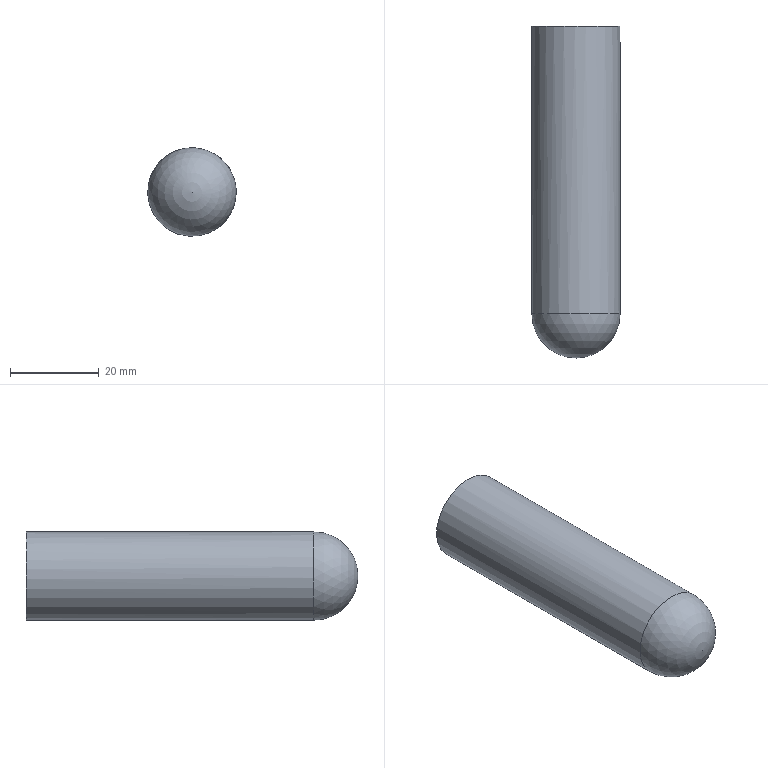Component | NX | PLUNGER_2 | 1 solid | 5 faces | box 20 x 75 x 20 mm | volume 9446 mm3 | cylinder 2 | plane 2 | sphere 1 | commonest cylinder face diameters 20 x1 16 x1
STEP:
#1=CARTESIAN_POINT('',(0.,0.,0.));
#2=DIRECTION('',(0.,0.,1.));
#3=DIRECTION('',(1.,0.,0.));
#4=AXIS2_PLACEMENT_3D('',#1,#2,#3);
#5=CARTESIAN_POINT('',(-34.641,119.,-20.));
#6=VERTEX_POINT('',#5);
#7=CARTESIAN_POINT('',(-17.321,119.,-10.));
#8=VERTEX_POINT('',#7);
#9=CARTESIAN_POINT('',(-25.981,119.,-15.));
#10=DIRECTION('',(0.,1.,0.));
#11=DIRECTION('',(-0.866,0.,-0.5));
#12=AXIS2_PLACEMENT_3D('',#9,#10,#11);
#13=CIRCLE('',#12,10.);
#14=CARTESIAN_POINT('',(-25.981,109.,-15.));
#15=DIRECTION('',(0.,1.,0.));
#16=DIRECTION('',(-0.866,0.,-0.5));
#17=AXIS2_PLACEMENT_3D('',#14,#15,#16);
#18=CYLINDRICAL_SURFACE('',#17,10.);
#19=CARTESIAN_POINT('',(0.,10.));
#20=DIRECTION('',(1.,0.));
#21=VECTOR('',#20,1.);
#22=LINE('',#19,#21);
#23=(GEOMETRIC_REPRESENTATION_CONTEXT(2)PARAMETRIC_REPRESENTATION_CONTEXT()REPRESENTATION_CONTEXT('',''));
#24=DEFINITIONAL_REPRESENTATION('',(#22),#23);
#25=PCURVE('',#18,#24);
#26=CARTESIAN_POINT('',(-25.981,119.,-15.));
#27=DIRECTION('',(0.,-1.,0.));
#28=DIRECTION('',(0.866,0.,0.5));
#29=AXIS2_PLACEMENT_3D('',#26,#27,#28);
#30=SPHERICAL_SURFACE('',#29,10.);
#31=CARTESIAN_POINT('',(3.142,0.));
#32=CARTESIAN_POINT('',(3.046,0.));
#33=CARTESIAN_POINT('',(2.856,0.));
#34=CARTESIAN_POINT('',(2.57,0.));
#35=CARTESIAN_POINT('',(2.285,0.));
#36=CARTESIAN_POINT('',(1.999,0.));
#37=CARTESIAN_POINT('',(1.714,0.));
#38=CARTESIAN_POINT('',(1.428,0.));
#39=CARTESIAN_POINT('',(1.142,0.));
#40=CARTESIAN_POINT('',(0.8568,0.));
#41=CARTESIAN_POINT('',(0.5712,0.));
#42=CARTESIAN_POINT('',(0.2856,0.));
#43=CARTESIAN_POINT('',(0.,0.));
#44=CARTESIAN_POINT('',(-0.2856,0.));
#45=CARTESIAN_POINT('',(-0.5712,0.));
#46=CARTESIAN_POINT('',(-0.8568,0.));
#47=CARTESIAN_POINT('',(-1.142,0.));
#48=CARTESIAN_POINT('',(-1.428,0.));
#49=CARTESIAN_POINT('',(-1.714,0.));
#50=CARTESIAN_POINT('',(-1.999,0.));
#51=CARTESIAN_POINT('',(-2.285,0.));
#52=CARTESIAN_POINT('',(-2.57,0.));
#53=CARTESIAN_POINT('',(-2.856,0.));
#54=CARTESIAN_POINT('',(-3.046,0.));
#55=CARTESIAN_POINT('',(-3.142,0.));
#56=B_SPLINE_CURVE_WITH_KNOTS('',3,(#31,#32,#33,#34,#35,#36,#37,#38,#39,#40,#41,#42,#43,#44,#45,#46,#47,#48,#49,#50,#51,#52,#53,#54,#55),.UNSPECIFIED.,.F.,.F.,(4,1,1,1,1,1,1,1,1,1,1,1,1,1,1,1,1,1,1,1,1,1,4),(0.,0.2856,0.5712,0.8568,1.142,1.428,1.714,1.999,2.285,2.57,2.856,3.142,3.427,3.713,3.998,4.284,4.57,4.855,5.141,5.426,5.712,5.998,6.283),.QUASI_UNIFORM_KNOTS.);
#57=(GEOMETRIC_REPRESENTATION_CONTEXT(2)PARAMETRIC_REPRESENTATION_CONTEXT()REPRESENTATION_CONTEXT('',''));
#58=DEFINITIONAL_REPRESENTATION('',(#56),#57);
#59=PCURVE('',#30,#58);
#60=SURFACE_CURVE('',#13,(#25,#59),.PCURVE_S1.);
#61=EDGE_CURVE('',#6,#8,#60,.T.);
#62=ORIENTED_EDGE('',*,*,#61,.T.);
#63=CARTESIAN_POINT('',(-25.981,119.,-15.));
#64=DIRECTION('',(0.,1.,0.));
#65=DIRECTION('',(-0.866,0.,-0.5));
#66=AXIS2_PLACEMENT_3D('',#63,#64,#65);
#67=CIRCLE('',#66,10.);
#68=CARTESIAN_POINT('',(0.,10.));
#69=DIRECTION('',(1.,0.));
#70=VECTOR('',#69,1.);
#71=LINE('',#68,#70);
#72=(GEOMETRIC_REPRESENTATION_CONTEXT(2)PARAMETRIC_REPRESENTATION_CONTEXT()REPRESENTATION_CONTEXT('',''));
#73=DEFINITIONAL_REPRESENTATION('',(#71),#72);
#74=PCURVE('',#18,#73);
#75=CARTESIAN_POINT('',(9.425,0.));
#76=CARTESIAN_POINT('',(9.33,0.));
#77=CARTESIAN_POINT('',(9.139,0.));
#78=CARTESIAN_POINT('',(8.854,0.));
#79=CARTESIAN_POINT('',(8.568,0.));
#80=CARTESIAN_POINT('',(8.282,0.));
#81=CARTESIAN_POINT('',(7.997,0.));
#82=CARTESIAN_POINT('',(7.711,0.));
#83=CARTESIAN_POINT('',(7.426,0.));
#84=CARTESIAN_POINT('',(7.14,0.));
#85=CARTESIAN_POINT('',(6.854,0.));
#86=CARTESIAN_POINT('',(6.569,0.));
#87=CARTESIAN_POINT('',(6.283,0.));
#88=CARTESIAN_POINT('',(5.998,0.));
#89=CARTESIAN_POINT('',(5.712,0.));
#90=CARTESIAN_POINT('',(5.426,0.));
#91=CARTESIAN_POINT('',(5.141,0.));
#92=CARTESIAN_POINT('',(4.855,0.));
#93=CARTESIAN_POINT('',(4.57,0.));
#94=CARTESIAN_POINT('',(4.284,0.));
#95=CARTESIAN_POINT('',(3.998,0.));
#96=CARTESIAN_POINT('',(3.713,0.));
#97=CARTESIAN_POINT('',(3.427,0.));
#98=CARTESIAN_POINT('',(3.237,0.));
#99=CARTESIAN_POINT('',(3.142,0.));
#100=B_SPLINE_CURVE_WITH_KNOTS('',3,(#75,#76,#77,#78,#79,#80,#81,#82,#83,#84,#85,#86,#87,#88,#89,#90,#91,#92,#93,#94,#95,#96,#97,#98,#99),.UNSPECIFIED.,.F.,.F.,(4,1,1,1,1,1,1,1,1,1,1,1,1,1,1,1,1,1,1,1,1,1,4),(0.,0.2856,0.5712,0.8568,1.142,1.428,1.714,1.999,2.285,2.57,2.856,3.142,3.427,3.713,3.998,4.284,4.57,4.855,5.141,5.426,5.712,5.998,6.283),.QUASI_UNIFORM_KNOTS.);
#101=(GEOMETRIC_REPRESENTATION_CONTEXT(2)PARAMETRIC_REPRESENTATION_CONTEXT()REPRESENTATION_CONTEXT('',''));
#102=DEFINITIONAL_REPRESENTATION('',(#100),#101);
#103=PCURVE('',#30,#102);
#104=SURFACE_CURVE('',#67,(#74,#103),.PCURVE_S1.);
#105=EDGE_CURVE('',#8,#6,#104,.T.);
#106=ORIENTED_EDGE('',*,*,#105,.T.);
#107=CARTESIAN_POINT('',(-34.641,184.,-20.));
#108=VERTEX_POINT('',#107);
#109=CARTESIAN_POINT('',(-34.641,119.,-20.));
#110=CARTESIAN_POINT('',(-34.641,184.,-20.));
#111=B_SPLINE_CURVE_WITH_KNOTS('',1,(#109,#110),.UNSPECIFIED.,.F.,.F.,(2,2),(10.,75.),.PIECEWISE_BEZIER_KNOTS.);
#112=CARTESIAN_POINT('',(6.283,0.));
#113=DIRECTION('',(0.,1.));
#114=VECTOR('',#113,1.);
#115=LINE('',#112,#114);
#116=(GEOMETRIC_REPRESENTATION_CONTEXT(2)PARAMETRIC_REPRESENTATION_CONTEXT()REPRESENTATION_CONTEXT('',''));
#117=DEFINITIONAL_REPRESENTATION('',(#115),#116);
#118=PCURVE('',#18,#117);
#119=CARTESIAN_POINT('',(0.,0.));
#120=DIRECTION('',(0.,1.));
#121=VECTOR('',#120,1.);
#122=LINE('',#119,#121);
#123=(GEOMETRIC_REPRESENTATION_CONTEXT(2)PARAMETRIC_REPRESENTATION_CONTEXT()REPRESENTATION_CONTEXT('',''));
#124=DEFINITIONAL_REPRESENTATION('',(#122),#123);
#125=PCURVE('',#18,#124);
#126=SEAM_CURVE('',#111,(#118,#125),.PCURVE_S1.);
#127=EDGE_CURVE('',#6,#108,#126,.T.);
#128=ORIENTED_EDGE('',*,*,#127,.T.);
#129=CARTESIAN_POINT('',(-30.981,184.,-6.34));
#130=VERTEX_POINT('',#129);
#131=CARTESIAN_POINT('',(-25.981,184.,-15.));
#132=DIRECTION('',(0.,-1.,0.));
#133=DIRECTION('',(-0.5,0.,0.866));
#134=AXIS2_PLACEMENT_3D('',#131,#132,#133);
#135=CIRCLE('',#134,10.);
#136=CARTESIAN_POINT('',(7.854,75.));
#137=DIRECTION('',(-1.,0.));
#138=VECTOR('',#137,1.);
#139=LINE('',#136,#138);
#140=(GEOMETRIC_REPRESENTATION_CONTEXT(2)PARAMETRIC_REPRESENTATION_CONTEXT()REPRESENTATION_CONTEXT('',''));
#141=DEFINITIONAL_REPRESENTATION('',(#139),#140);
#142=PCURVE('',#18,#141);
#143=CARTESIAN_POINT('',(-25.981,184.,-15.));
#144=DIRECTION('',(0.,-1.,0.));
#145=DIRECTION('',(0.866,0.,0.5));
#146=AXIS2_PLACEMENT_3D('',#143,#144,#145);
#147=PLANE('',#146);
#148=CARTESIAN_POINT('',(0.,0.));
#149=DIRECTION('',(0.,1.));
#150=AXIS2_PLACEMENT_2D('',#148,#149);
#151=CIRCLE('',#150,10.);
#152=(GEOMETRIC_REPRESENTATION_CONTEXT(2)PARAMETRIC_REPRESENTATION_CONTEXT()REPRESENTATION_CONTEXT('',''));
#153=DEFINITIONAL_REPRESENTATION('',(#151),#152);
#154=PCURVE('',#147,#153);
#155=SURFACE_CURVE('',#135,(#142,#154),.PCURVE_S1.);
#156=EDGE_CURVE('',#108,#130,#155,.T.);
#157=ORIENTED_EDGE('',*,*,#156,.T.);
#158=CARTESIAN_POINT('',(-25.981,184.,-15.));
#159=DIRECTION('',(0.,-1.,0.));
#160=DIRECTION('',(-0.5,0.,0.866));
#161=AXIS2_PLACEMENT_3D('',#158,#159,#160);
#162=CIRCLE('',#161,10.);
#163=CARTESIAN_POINT('',(1.571,75.));
#164=DIRECTION('',(-1.,0.));
#165=VECTOR('',#164,1.);
#166=LINE('',#163,#165);
#167=(GEOMETRIC_REPRESENTATION_CONTEXT(2)PARAMETRIC_REPRESENTATION_CONTEXT()REPRESENTATION_CONTEXT('',''));
#168=DEFINITIONAL_REPRESENTATION('',(#166),#167);
#169=PCURVE('',#18,#168);
#170=CARTESIAN_POINT('',(0.,0.));
#171=DIRECTION('',(0.,1.));
#172=AXIS2_PLACEMENT_2D('',#170,#171);
#173=CIRCLE('',#172,10.);
#174=(GEOMETRIC_REPRESENTATION_CONTEXT(2)PARAMETRIC_REPRESENTATION_CONTEXT()REPRESENTATION_CONTEXT('',''));
#175=DEFINITIONAL_REPRESENTATION('',(#173),#174);
#176=PCURVE('',#147,#175);
#177=SURFACE_CURVE('',#162,(#169,#176),.PCURVE_S1.);
#178=EDGE_CURVE('',#130,#108,#177,.T.);
#179=ORIENTED_EDGE('',*,*,#178,.T.);
#180=ORIENTED_EDGE('',*,*,#127,.F.);
#181=EDGE_LOOP('',(#62,#106,#128,#157,#179,#180));
#182=FACE_BOUND('',#181,.T.);
#183=ADVANCED_FACE('',(#182),#18,.T.);
#184=CARTESIAN_POINT('',(-19.053,184.,-11.));
#185=VERTEX_POINT('',#184);
#186=CARTESIAN_POINT('',(-25.981,184.,-15.));
#187=DIRECTION('',(0.,-1.,0.));
#188=DIRECTION('',(0.866,0.,0.5));
#189=AXIS2_PLACEMENT_3D('',#186,#187,#188);
#190=CIRCLE('',#189,8.);
#191=CARTESIAN_POINT('',(0.,0.));
#192=DIRECTION('',(1.,0.));
#193=AXIS2_PLACEMENT_2D('',#191,#192);
#194=CIRCLE('',#193,8.);
#195=(GEOMETRIC_REPRESENTATION_CONTEXT(2)PARAMETRIC_REPRESENTATION_CONTEXT()REPRESENTATION_CONTEXT('',''));
#196=DEFINITIONAL_REPRESENTATION('',(#194),#195);
#197=PCURVE('',#147,#196);
#198=CARTESIAN_POINT('',(-25.981,184.,-15.));
#199=DIRECTION('',(0.,-1.,0.));
#200=DIRECTION('',(0.866,0.,0.5));
#201=AXIS2_PLACEMENT_3D('',#198,#199,#200);
#202=CYLINDRICAL_SURFACE('',#201,8.);
#203=CARTESIAN_POINT('',(0.,0.));
#204=DIRECTION('',(1.,0.));
#205=VECTOR('',#204,1.);
#206=LINE('',#203,#205);
#207=(GEOMETRIC_REPRESENTATION_CONTEXT(2)PARAMETRIC_REPRESENTATION_CONTEXT()REPRESENTATION_CONTEXT('',''));
#208=DEFINITIONAL_REPRESENTATION('',(#206),#207);
#209=PCURVE('',#202,#208);
#210=SURFACE_CURVE('',#190,(#197,#209),.PCURVE_S1.);
#211=EDGE_CURVE('',#185,#185,#210,.T.);
#212=ORIENTED_EDGE('',*,*,#211,.T.);
#213=EDGE_LOOP('',(#212));
#214=FACE_BOUND('',#213,.T.);
#215=ORIENTED_EDGE('',*,*,#178,.F.);
#216=ORIENTED_EDGE('',*,*,#156,.F.);
#217=EDGE_LOOP('',(#215,#216));
#218=FACE_BOUND('',#217,.T.);
#219=ADVANCED_FACE('',(#214,#218),#147,.F.);
#220=ORIENTED_EDGE('',*,*,#105,.F.);
#221=CARTESIAN_POINT('',(-25.981,109.,-15.));
#222=VERTEX_POINT('',#221);
#223=CARTESIAN_POINT('',(-17.321,119.,-10.));
#224=CARTESIAN_POINT('',(-17.321,116.756,-10.));
#225=CARTESIAN_POINT('',(-17.829,114.512,-10.294));
#226=CARTESIAN_POINT('',(-18.847,112.453,-10.881));
#227=CARTESIAN_POINT('',(-20.31,110.762,-11.726));
#228=CARTESIAN_POINT('',(-22.094,109.587,-12.756));
#229=CARTESIAN_POINT('',(-24.037,109.,-13.878));
#230=CARTESIAN_POINT('',(-25.981,109.,-15.));
#231=B_SPLINE_CURVE_WITH_KNOTS('',7,(#223,#224,#225,#226,#227,#228,#229,#230),.UNSPECIFIED.,.F.,.F.,(8,8),(0.,1.571),.PIECEWISE_BEZIER_KNOTS.);
#232=CARTESIAN_POINT('',(6.283,0.));
#233=DIRECTION('',(0.,1.));
#234=VECTOR('',#233,1.);
#235=LINE('',#232,#234);
#236=(GEOMETRIC_REPRESENTATION_CONTEXT(2)PARAMETRIC_REPRESENTATION_CONTEXT()REPRESENTATION_CONTEXT('',''));
#237=DEFINITIONAL_REPRESENTATION('',(#235),#236);
#238=PCURVE('',#30,#237);
#239=CARTESIAN_POINT('',(0.,0.));
#240=DIRECTION('',(0.,1.));
#241=VECTOR('',#240,1.);
#242=LINE('',#239,#241);
#243=(GEOMETRIC_REPRESENTATION_CONTEXT(2)PARAMETRIC_REPRESENTATION_CONTEXT()REPRESENTATION_CONTEXT('',''));
#244=DEFINITIONAL_REPRESENTATION('',(#242),#243);
#245=PCURVE('',#30,#244);
#246=SEAM_CURVE('',#231,(#238,#245),.PCURVE_S1.);
#247=EDGE_CURVE('',#8,#222,#246,.T.);
#248=ORIENTED_EDGE('',*,*,#247,.T.);
#249=ORIENTED_EDGE('',*,*,#247,.F.);
#250=ORIENTED_EDGE('',*,*,#61,.F.);
#251=EDGE_LOOP('',(#220,#248,#249,#250));
#252=FACE_BOUND('',#251,.T.);
#253=ADVANCED_FACE('',(#252),#30,.T.);
#254=CARTESIAN_POINT('',(-19.053,119.,-11.));
#255=VERTEX_POINT('',#254);
#256=CARTESIAN_POINT('',(-25.981,119.,-15.));
#257=DIRECTION('',(0.,1.,0.));
#258=DIRECTION('',(0.866,0.,0.5));
#259=AXIS2_PLACEMENT_3D('',#256,#257,#258);
#260=CIRCLE('',#259,8.);
#261=CARTESIAN_POINT('',(-25.981,119.,-15.));
#262=DIRECTION('',(0.,-1.,0.));
#263=DIRECTION('',(0.866,0.,0.5));
#264=AXIS2_PLACEMENT_3D('',#261,#262,#263);
#265=PLANE('',#264);
#266=CARTESIAN_POINT('',(8.,0.));
#267=CARTESIAN_POINT('',(8.,-13.856));
#268=CARTESIAN_POINT('',(-4.,-6.928));
#269=CARTESIAN_POINT('',(-16.,-0.));
#270=CARTESIAN_POINT('',(-4.,6.928));
#271=CARTESIAN_POINT('',(8.,13.856));
#272=CARTESIAN_POINT('',(8.,0.));
#273=(BOUNDED_CURVE()B_SPLINE_CURVE(2,(#266,#267,#268,#269,#270,#271,#272),.UNSPECIFIED.,.T.,.F.)B_SPLINE_CURVE_WITH_KNOTS((1,2,2,2,2,1),(-2.094,0.,2.094,4.189,6.283,8.378),.UNSPECIFIED.)CURVE()GEOMETRIC_REPRESENTATION_ITEM()RATIONAL_B_SPLINE_CURVE((1.,0.5,1.,0.5,1.,0.5,1.))REPRESENTATION_ITEM(''));
#274=(GEOMETRIC_REPRESENTATION_CONTEXT(2)PARAMETRIC_REPRESENTATION_CONTEXT()REPRESENTATION_CONTEXT('',''));
#275=DEFINITIONAL_REPRESENTATION('',(#273),#274);
#276=PCURVE('',#265,#275);
#277=CARTESIAN_POINT('',(6.283,65.));
#278=DIRECTION('',(-1.,0.));
#279=VECTOR('',#278,1.);
#280=LINE('',#277,#279);
#281=(GEOMETRIC_REPRESENTATION_CONTEXT(2)PARAMETRIC_REPRESENTATION_CONTEXT()REPRESENTATION_CONTEXT('',''));
#282=DEFINITIONAL_REPRESENTATION('',(#280),#281);
#283=PCURVE('',#202,#282);
#284=SURFACE_CURVE('',#260,(#276,#283),.PCURVE_S1.);
#285=EDGE_CURVE('',#255,#255,#284,.T.);
#286=ORIENTED_EDGE('',*,*,#285,.T.);
#287=EDGE_LOOP('',(#286));
#288=FACE_BOUND('',#287,.T.);
#289=ADVANCED_FACE('',(#288),#265,.F.);
#290=ORIENTED_EDGE('',*,*,#285,.T.);
#291=CARTESIAN_POINT('',(-19.053,184.,-11.));
#292=CARTESIAN_POINT('',(-19.053,119.,-11.));
#293=B_SPLINE_CURVE_WITH_KNOTS('',1,(#291,#292),.UNSPECIFIED.,.F.,.F.,(2,2),(0.,65.),.PIECEWISE_BEZIER_KNOTS.);
#294=CARTESIAN_POINT('',(0.,0.));
#295=DIRECTION('',(0.,1.));
#296=VECTOR('',#295,1.);
#297=LINE('',#294,#296);
#298=(GEOMETRIC_REPRESENTATION_CONTEXT(2)PARAMETRIC_REPRESENTATION_CONTEXT()REPRESENTATION_CONTEXT('',''));
#299=DEFINITIONAL_REPRESENTATION('',(#297),#298);
#300=PCURVE('',#202,#299);
#301=CARTESIAN_POINT('',(6.283,0.));
#302=DIRECTION('',(0.,1.));
#303=VECTOR('',#302,1.);
#304=LINE('',#301,#303);
#305=(GEOMETRIC_REPRESENTATION_CONTEXT(2)PARAMETRIC_REPRESENTATION_CONTEXT()REPRESENTATION_CONTEXT('',''));
#306=DEFINITIONAL_REPRESENTATION('',(#304),#305);
#307=PCURVE('',#202,#306);
#308=SEAM_CURVE('',#293,(#300,#307),.PCURVE_S1.);
#309=EDGE_CURVE('',#185,#255,#308,.T.);
#310=ORIENTED_EDGE('',*,*,#309,.F.);
#311=ORIENTED_EDGE('',*,*,#211,.T.);
#312=ORIENTED_EDGE('',*,*,#309,.T.);
#313=EDGE_LOOP('',(#290,#310,#311,#312));
#314=FACE_BOUND('',#313,.F.);
#315=ADVANCED_FACE('',(#314),#202,.F.);
#316=CLOSED_SHELL('',(#183,#219,#253,#289,#315));
#317=MANIFOLD_SOLID_BREP('',#316);
#318=(LENGTH_UNIT()NAMED_UNIT(*)SI_UNIT(.MILLI.,.METRE.));
#319=UNCERTAINTY_MEASURE_WITH_UNIT(LENGTH_MEASURE(0.000005),#318,'','');
#320=(NAMED_UNIT(*)PLANE_ANGLE_UNIT()SI_UNIT($,.RADIAN.));
#321=(NAMED_UNIT(*)SI_UNIT($,.STERADIAN.)SOLID_ANGLE_UNIT());
#322=(GEOMETRIC_REPRESENTATION_CONTEXT(3)GLOBAL_UNCERTAINTY_ASSIGNED_CONTEXT((#319))GLOBAL_UNIT_ASSIGNED_CONTEXT((#318,#320,#321))REPRESENTATION_CONTEXT('',''));
#323=ADVANCED_BREP_SHAPE_REPRESENTATION('',(#4,#317),#322);